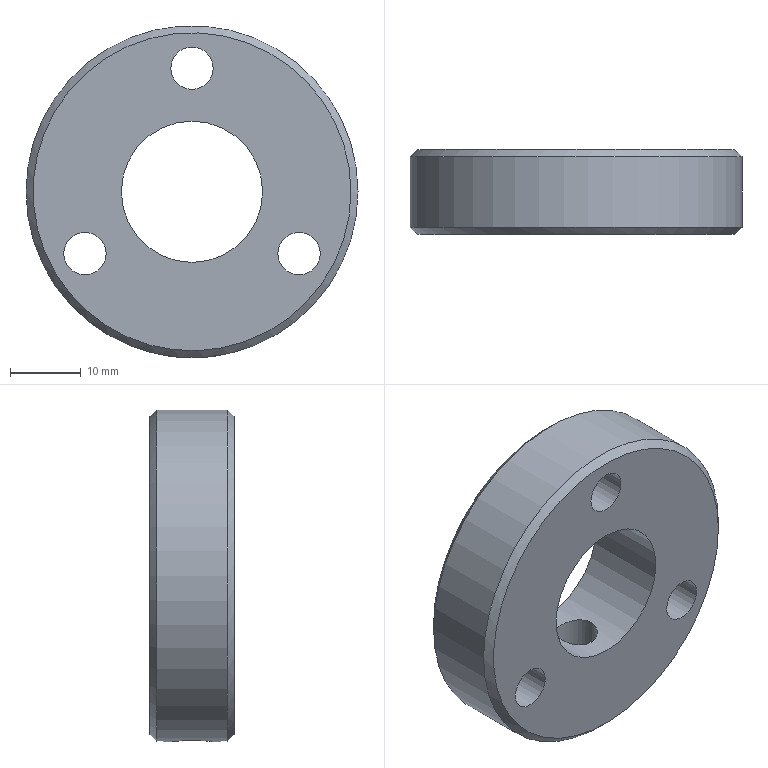Component | NX | 9_SPACER | 1 solid | 10 faces | volume 15503 mm3 | cylinder 6 | plane 2 | cone 2 | commonest cylinder face diameters 6 x4 47 x1 20 x1